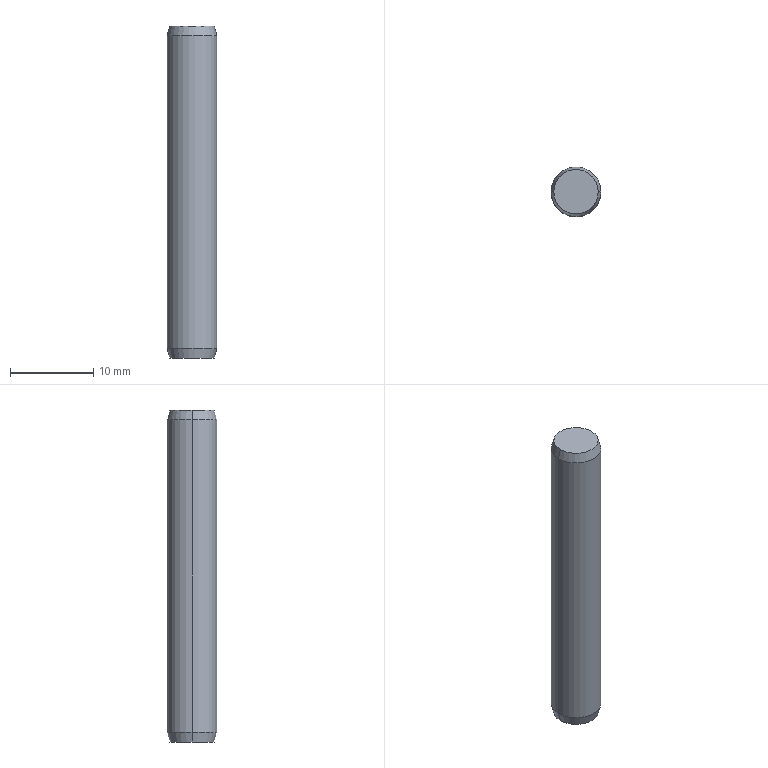Component | NX | GB_T_119_1_2000_CYLINDRICALPIN_6X40 | 1 solid | 8 faces | box 6 x 6 x 40 mm | volume 1124 mm3 | cone 4 | cylinder 2 | plane 2 | commonest cylinder face diameters 6 x2
STEP:
#1=CARTESIAN_POINT('',(0.,0.,0.));
#2=DIRECTION('',(0.,0.,1.));
#3=DIRECTION('',(1.,0.,0.));
#4=AXIS2_PLACEMENT_3D('',#1,#2,#3);
#5=CARTESIAN_POINT('',(7.514,-108.,34.));
#6=VERTEX_POINT('',#5);
#7=CARTESIAN_POINT('',(2.157,-108.,34.));
#8=VERTEX_POINT('',#7);
#9=CARTESIAN_POINT('',(4.835,-108.,34.));
#10=DIRECTION('',(0.,0.,1.));
#11=DIRECTION('',(1.,0.,0.));
#12=AXIS2_PLACEMENT_3D('',#9,#10,#11);
#13=CIRCLE('',#12,2.678);
#14=CARTESIAN_POINT('',(4.835,-108.,35.2));
#15=DIRECTION('',(0.,0.,1.));
#16=DIRECTION('',(-1.,0.,0.));
#17=AXIS2_PLACEMENT_3D('',#14,#15,#16);
#18=CONICAL_SURFACE('',#17,3.,0.2618);
#19=CARTESIAN_POINT('',(3.142,-1.2));
#20=DIRECTION('',(1.,0.));
#21=VECTOR('',#20,1.);
#22=LINE('',#19,#21);
#23=(GEOMETRIC_REPRESENTATION_CONTEXT(2)PARAMETRIC_REPRESENTATION_CONTEXT()REPRESENTATION_CONTEXT('',''));
#24=DEFINITIONAL_REPRESENTATION('',(#22),#23);
#25=PCURVE('',#18,#24);
#26=CARTESIAN_POINT('',(4.835,-105.322,34.));
#27=DIRECTION('',(0.,0.,-1.));
#28=DIRECTION('',(1.,0.,0.));
#29=AXIS2_PLACEMENT_3D('',#26,#27,#28);
#30=PLANE('',#29);
#31=CARTESIAN_POINT('',(2.678,2.678));
#32=CARTESIAN_POINT('',(2.678,-1.961));
#33=CARTESIAN_POINT('',(-1.339,0.3588));
#34=CARTESIAN_POINT('',(-5.357,2.678));
#35=CARTESIAN_POINT('',(-1.339,4.998));
#36=CARTESIAN_POINT('',(2.678,7.318));
#37=CARTESIAN_POINT('',(2.678,2.678));
#38=(BOUNDED_CURVE()B_SPLINE_CURVE(2,(#31,#32,#33,#34,#35,#36,#37),.UNSPECIFIED.,.T.,.F.)B_SPLINE_CURVE_WITH_KNOTS((1,2,2,2,2,1),(-2.094,0.,2.094,4.189,6.283,8.378),.UNSPECIFIED.)CURVE()GEOMETRIC_REPRESENTATION_ITEM()RATIONAL_B_SPLINE_CURVE((1.,0.5,1.,0.5,1.,0.5,1.))REPRESENTATION_ITEM(''));
#39=(GEOMETRIC_REPRESENTATION_CONTEXT(2)PARAMETRIC_REPRESENTATION_CONTEXT()REPRESENTATION_CONTEXT('',''));
#40=DEFINITIONAL_REPRESENTATION('',(#38),#39);
#41=PCURVE('',#30,#40);
#42=SURFACE_CURVE('',#13,(#25,#41),.PCURVE_S1.);
#43=EDGE_CURVE('',#6,#8,#42,.T.);
#44=ORIENTED_EDGE('',*,*,#43,.T.);
#45=CARTESIAN_POINT('',(1.835,-108.,35.2));
#46=VERTEX_POINT('',#45);
#47=CARTESIAN_POINT('',(1.835,-108.,35.2));
#48=DIRECTION('',(-0.2588,0.,0.9659));
#49=VECTOR('',#48,1.);
#50=LINE('',#47,#49);
#51=CARTESIAN_POINT('',(6.283,-0.));
#52=DIRECTION('',(0.,1.));
#53=VECTOR('',#52,1.);
#54=LINE('',#51,#53);
#55=(GEOMETRIC_REPRESENTATION_CONTEXT(2)PARAMETRIC_REPRESENTATION_CONTEXT()REPRESENTATION_CONTEXT('',''));
#56=DEFINITIONAL_REPRESENTATION('',(#54),#55);
#57=PCURVE('',#18,#56);
#58=CARTESIAN_POINT('',(4.835,-108.,35.2));
#59=DIRECTION('',(0.,0.,1.));
#60=DIRECTION('',(-1.,0.,0.));
#61=AXIS2_PLACEMENT_3D('',#58,#59,#60);
#62=CONICAL_SURFACE('',#61,3.,0.2618);
#63=CARTESIAN_POINT('',(0.,-0.));
#64=DIRECTION('',(0.,1.));
#65=VECTOR('',#64,1.);
#66=LINE('',#63,#65);
#67=(GEOMETRIC_REPRESENTATION_CONTEXT(2)PARAMETRIC_REPRESENTATION_CONTEXT()REPRESENTATION_CONTEXT('',''));
#68=DEFINITIONAL_REPRESENTATION('',(#66),#67);
#69=PCURVE('',#62,#68);
#70=SURFACE_CURVE('',#50,(#57,#69),.PCURVE_S1.);
#71=EDGE_CURVE('',#8,#46,#70,.T.);
#72=ORIENTED_EDGE('',*,*,#71,.T.);
#73=CARTESIAN_POINT('',(7.835,-108.,35.2));
#74=VERTEX_POINT('',#73);
#75=CARTESIAN_POINT('',(4.835,-108.,35.2));
#76=DIRECTION('',(0.,0.,1.));
#77=DIRECTION('',(1.,0.,0.));
#78=AXIS2_PLACEMENT_3D('',#75,#76,#77);
#79=CIRCLE('',#78,3.);
#80=CARTESIAN_POINT('',(3.142,0.));
#81=DIRECTION('',(1.,0.));
#82=VECTOR('',#81,1.);
#83=LINE('',#80,#82);
#84=(GEOMETRIC_REPRESENTATION_CONTEXT(2)PARAMETRIC_REPRESENTATION_CONTEXT()REPRESENTATION_CONTEXT('',''));
#85=DEFINITIONAL_REPRESENTATION('',(#83),#84);
#86=PCURVE('',#18,#85);
#87=CARTESIAN_POINT('',(4.835,-108.,34.));
#88=DIRECTION('',(0.,0.,1.));
#89=DIRECTION('',(-1.,0.,0.));
#90=AXIS2_PLACEMENT_3D('',#87,#88,#89);
#91=CYLINDRICAL_SURFACE('',#90,3.);
#92=CARTESIAN_POINT('',(3.142,1.2));
#93=DIRECTION('',(1.,0.));
#94=VECTOR('',#93,1.);
#95=LINE('',#92,#94);
#96=(GEOMETRIC_REPRESENTATION_CONTEXT(2)PARAMETRIC_REPRESENTATION_CONTEXT()REPRESENTATION_CONTEXT('',''));
#97=DEFINITIONAL_REPRESENTATION('',(#95),#96);
#98=PCURVE('',#91,#97);
#99=SURFACE_CURVE('',#79,(#86,#98),.PCURVE_S1.);
#100=EDGE_CURVE('',#74,#46,#99,.T.);
#101=ORIENTED_EDGE('',*,*,#100,.F.);
#102=CARTESIAN_POINT('',(7.835,-108.,35.2));
#103=DIRECTION('',(0.2588,0.,0.9659));
#104=VECTOR('',#103,1.);
#105=LINE('',#102,#104);
#106=CARTESIAN_POINT('',(3.142,-0.));
#107=DIRECTION('',(0.,1.));
#108=VECTOR('',#107,1.);
#109=LINE('',#106,#108);
#110=(GEOMETRIC_REPRESENTATION_CONTEXT(2)PARAMETRIC_REPRESENTATION_CONTEXT()REPRESENTATION_CONTEXT('',''));
#111=DEFINITIONAL_REPRESENTATION('',(#109),#110);
#112=PCURVE('',#18,#111);
#113=CARTESIAN_POINT('',(3.142,-0.));
#114=DIRECTION('',(0.,1.));
#115=VECTOR('',#114,1.);
#116=LINE('',#113,#115);
#117=(GEOMETRIC_REPRESENTATION_CONTEXT(2)PARAMETRIC_REPRESENTATION_CONTEXT()REPRESENTATION_CONTEXT('',''));
#118=DEFINITIONAL_REPRESENTATION('',(#116),#117);
#119=PCURVE('',#62,#118);
#120=SURFACE_CURVE('',#105,(#112,#119),.PCURVE_S1.);
#121=EDGE_CURVE('',#6,#74,#120,.T.);
#122=ORIENTED_EDGE('',*,*,#121,.F.);
#123=EDGE_LOOP('',(#44,#72,#101,#122));
#124=FACE_BOUND('',#123,.T.);
#125=ADVANCED_FACE('',(#124),#18,.T.);
#126=ORIENTED_EDGE('',*,*,#100,.T.);
#127=CARTESIAN_POINT('',(1.835,-108.,72.8));
#128=VERTEX_POINT('',#127);
#129=CARTESIAN_POINT('',(1.835,-108.,34.));
#130=DIRECTION('',(0.,0.,1.));
#131=VECTOR('',#130,1.);
#132=LINE('',#129,#131);
#133=CARTESIAN_POINT('',(6.283,0.));
#134=DIRECTION('',(0.,1.));
#135=VECTOR('',#134,1.);
#136=LINE('',#133,#135);
#137=(GEOMETRIC_REPRESENTATION_CONTEXT(2)PARAMETRIC_REPRESENTATION_CONTEXT()REPRESENTATION_CONTEXT('',''));
#138=DEFINITIONAL_REPRESENTATION('',(#136),#137);
#139=PCURVE('',#91,#138);
#140=CARTESIAN_POINT('',(4.835,-108.,34.));
#141=DIRECTION('',(0.,0.,1.));
#142=DIRECTION('',(-1.,0.,0.));
#143=AXIS2_PLACEMENT_3D('',#140,#141,#142);
#144=CYLINDRICAL_SURFACE('',#143,3.);
#145=CARTESIAN_POINT('',(0.,0.));
#146=DIRECTION('',(0.,1.));
#147=VECTOR('',#146,1.);
#148=LINE('',#145,#147);
#149=(GEOMETRIC_REPRESENTATION_CONTEXT(2)PARAMETRIC_REPRESENTATION_CONTEXT()REPRESENTATION_CONTEXT('',''));
#150=DEFINITIONAL_REPRESENTATION('',(#148),#149);
#151=PCURVE('',#144,#150);
#152=SURFACE_CURVE('',#132,(#139,#151),.PCURVE_S1.);
#153=EDGE_CURVE('',#46,#128,#152,.T.);
#154=ORIENTED_EDGE('',*,*,#153,.T.);
#155=CARTESIAN_POINT('',(7.835,-108.,72.8));
#156=VERTEX_POINT('',#155);
#157=CARTESIAN_POINT('',(4.835,-108.,72.8));
#158=DIRECTION('',(0.,0.,1.));
#159=DIRECTION('',(1.,0.,0.));
#160=AXIS2_PLACEMENT_3D('',#157,#158,#159);
#161=CIRCLE('',#160,3.);
#162=CARTESIAN_POINT('',(3.142,38.8));
#163=DIRECTION('',(1.,0.));
#164=VECTOR('',#163,1.);
#165=LINE('',#162,#164);
#166=(GEOMETRIC_REPRESENTATION_CONTEXT(2)PARAMETRIC_REPRESENTATION_CONTEXT()REPRESENTATION_CONTEXT('',''));
#167=DEFINITIONAL_REPRESENTATION('',(#165),#166);
#168=PCURVE('',#91,#167);
#169=CARTESIAN_POINT('',(4.835,-108.,74.));
#170=DIRECTION('',(0.,0.,-1.));
#171=DIRECTION('',(1.,0.,0.));
#172=AXIS2_PLACEMENT_3D('',#169,#170,#171);
#173=CONICAL_SURFACE('',#172,2.678,0.2618);
#174=CARTESIAN_POINT('',(6.283,1.2));
#175=DIRECTION('',(-1.,0.));
#176=VECTOR('',#175,1.);
#177=LINE('',#174,#176);
#178=(GEOMETRIC_REPRESENTATION_CONTEXT(2)PARAMETRIC_REPRESENTATION_CONTEXT()REPRESENTATION_CONTEXT('',''));
#179=DEFINITIONAL_REPRESENTATION('',(#177),#178);
#180=PCURVE('',#173,#179);
#181=SURFACE_CURVE('',#161,(#168,#180),.PCURVE_S1.);
#182=EDGE_CURVE('',#156,#128,#181,.T.);
#183=ORIENTED_EDGE('',*,*,#182,.F.);
#184=CARTESIAN_POINT('',(7.835,-108.,34.));
#185=DIRECTION('',(0.,0.,1.));
#186=VECTOR('',#185,1.);
#187=LINE('',#184,#186);
#188=CARTESIAN_POINT('',(3.142,0.));
#189=DIRECTION('',(0.,1.));
#190=VECTOR('',#189,1.);
#191=LINE('',#188,#190);
#192=(GEOMETRIC_REPRESENTATION_CONTEXT(2)PARAMETRIC_REPRESENTATION_CONTEXT()REPRESENTATION_CONTEXT('',''));
#193=DEFINITIONAL_REPRESENTATION('',(#191),#192);
#194=PCURVE('',#91,#193);
#195=CARTESIAN_POINT('',(3.142,0.));
#196=DIRECTION('',(0.,1.));
#197=VECTOR('',#196,1.);
#198=LINE('',#195,#197);
#199=(GEOMETRIC_REPRESENTATION_CONTEXT(2)PARAMETRIC_REPRESENTATION_CONTEXT()REPRESENTATION_CONTEXT('',''));
#200=DEFINITIONAL_REPRESENTATION('',(#198),#199);
#201=PCURVE('',#144,#200);
#202=SURFACE_CURVE('',#187,(#194,#201),.PCURVE_S1.);
#203=EDGE_CURVE('',#74,#156,#202,.T.);
#204=ORIENTED_EDGE('',*,*,#203,.F.);
#205=EDGE_LOOP('',(#126,#154,#183,#204));
#206=FACE_BOUND('',#205,.T.);
#207=ADVANCED_FACE('',(#206),#91,.T.);
#208=CARTESIAN_POINT('',(7.514,-108.,74.));
#209=VERTEX_POINT('',#208);
#210=CARTESIAN_POINT('',(2.157,-108.,74.));
#211=VERTEX_POINT('',#210);
#212=CARTESIAN_POINT('',(4.835,-108.,74.));
#213=DIRECTION('',(0.,0.,1.));
#214=DIRECTION('',(1.,0.,0.));
#215=AXIS2_PLACEMENT_3D('',#212,#213,#214);
#216=CIRCLE('',#215,2.678);
#217=CARTESIAN_POINT('',(6.283,0.));
#218=DIRECTION('',(-1.,0.));
#219=VECTOR('',#218,1.);
#220=LINE('',#217,#219);
#221=(GEOMETRIC_REPRESENTATION_CONTEXT(2)PARAMETRIC_REPRESENTATION_CONTEXT()REPRESENTATION_CONTEXT('',''));
#222=DEFINITIONAL_REPRESENTATION('',(#220),#221);
#223=PCURVE('',#173,#222);
#224=CARTESIAN_POINT('',(4.835,-105.322,74.));
#225=DIRECTION('',(0.,0.,1.));
#226=DIRECTION('',(-1.,0.,0.));
#227=AXIS2_PLACEMENT_3D('',#224,#225,#226);
#228=PLANE('',#227);
#229=CARTESIAN_POINT('',(0.,2.678));
#230=DIRECTION('',(-1.,0.));
#231=AXIS2_PLACEMENT_2D('',#229,#230);
#232=CIRCLE('',#231,2.678);
#233=(GEOMETRIC_REPRESENTATION_CONTEXT(2)PARAMETRIC_REPRESENTATION_CONTEXT()REPRESENTATION_CONTEXT('',''));
#234=DEFINITIONAL_REPRESENTATION('',(#232),#233);
#235=PCURVE('',#228,#234);
#236=SURFACE_CURVE('',#216,(#223,#235),.PCURVE_S1.);
#237=EDGE_CURVE('',#209,#211,#236,.T.);
#238=ORIENTED_EDGE('',*,*,#237,.F.);
#239=CARTESIAN_POINT('',(7.514,-108.,74.));
#240=DIRECTION('',(0.2588,0.,-0.9659));
#241=VECTOR('',#240,1.);
#242=LINE('',#239,#241);
#243=CARTESIAN_POINT('',(6.283,-0.));
#244=DIRECTION('',(0.,1.));
#245=VECTOR('',#244,1.);
#246=LINE('',#243,#245);
#247=(GEOMETRIC_REPRESENTATION_CONTEXT(2)PARAMETRIC_REPRESENTATION_CONTEXT()REPRESENTATION_CONTEXT('',''));
#248=DEFINITIONAL_REPRESENTATION('',(#246),#247);
#249=PCURVE('',#173,#248);
#250=CARTESIAN_POINT('',(4.835,-108.,74.));
#251=DIRECTION('',(0.,0.,-1.));
#252=DIRECTION('',(1.,0.,0.));
#253=AXIS2_PLACEMENT_3D('',#250,#251,#252);
#254=CONICAL_SURFACE('',#253,2.678,0.2618);
#255=CARTESIAN_POINT('',(0.,-0.));
#256=DIRECTION('',(0.,1.));
#257=VECTOR('',#256,1.);
#258=LINE('',#255,#257);
#259=(GEOMETRIC_REPRESENTATION_CONTEXT(2)PARAMETRIC_REPRESENTATION_CONTEXT()REPRESENTATION_CONTEXT('',''));
#260=DEFINITIONAL_REPRESENTATION('',(#258),#259);
#261=PCURVE('',#254,#260);
#262=SURFACE_CURVE('',#242,(#249,#261),.PCURVE_S1.);
#263=EDGE_CURVE('',#209,#156,#262,.T.);
#264=ORIENTED_EDGE('',*,*,#263,.T.);
#265=ORIENTED_EDGE('',*,*,#182,.T.);
#266=CARTESIAN_POINT('',(2.157,-108.,74.));
#267=DIRECTION('',(-0.2588,0.,-0.9659));
#268=VECTOR('',#267,1.);
#269=LINE('',#266,#268);
#270=CARTESIAN_POINT('',(3.142,0.));
#271=DIRECTION('',(0.,1.));
#272=VECTOR('',#271,1.);
#273=LINE('',#270,#272);
#274=(GEOMETRIC_REPRESENTATION_CONTEXT(2)PARAMETRIC_REPRESENTATION_CONTEXT()REPRESENTATION_CONTEXT('',''));
#275=DEFINITIONAL_REPRESENTATION('',(#273),#274);
#276=PCURVE('',#173,#275);
#277=CARTESIAN_POINT('',(3.142,0.));
#278=DIRECTION('',(0.,1.));
#279=VECTOR('',#278,1.);
#280=LINE('',#277,#279);
#281=(GEOMETRIC_REPRESENTATION_CONTEXT(2)PARAMETRIC_REPRESENTATION_CONTEXT()REPRESENTATION_CONTEXT('',''));
#282=DEFINITIONAL_REPRESENTATION('',(#280),#281);
#283=PCURVE('',#254,#282);
#284=SURFACE_CURVE('',#269,(#276,#283),.PCURVE_S1.);
#285=EDGE_CURVE('',#211,#128,#284,.T.);
#286=ORIENTED_EDGE('',*,*,#285,.F.);
#287=EDGE_LOOP('',(#238,#264,#265,#286));
#288=FACE_BOUND('',#287,.T.);
#289=ADVANCED_FACE('',(#288),#173,.T.);
#290=ORIENTED_EDGE('',*,*,#43,.F.);
#291=CARTESIAN_POINT('',(4.835,-108.,34.));
#292=DIRECTION('',(0.,0.,1.));
#293=DIRECTION('',(1.,0.,0.));
#294=AXIS2_PLACEMENT_3D('',#291,#292,#293);
#295=CIRCLE('',#294,2.678);
#296=CARTESIAN_POINT('',(2.678,2.678));
#297=CARTESIAN_POINT('',(2.678,-1.961));
#298=CARTESIAN_POINT('',(-1.339,0.3588));
#299=CARTESIAN_POINT('',(-5.357,2.678));
#300=CARTESIAN_POINT('',(-1.339,4.998));
#301=CARTESIAN_POINT('',(2.678,7.318));
#302=CARTESIAN_POINT('',(2.678,2.678));
#303=(BOUNDED_CURVE()B_SPLINE_CURVE(2,(#296,#297,#298,#299,#300,#301,#302),.UNSPECIFIED.,.T.,.F.)B_SPLINE_CURVE_WITH_KNOTS((1,2,2,2,2,1),(-2.094,0.,2.094,4.189,6.283,8.378),.UNSPECIFIED.)CURVE()GEOMETRIC_REPRESENTATION_ITEM()RATIONAL_B_SPLINE_CURVE((1.,0.5,1.,0.5,1.,0.5,1.))REPRESENTATION_ITEM(''));
#304=(GEOMETRIC_REPRESENTATION_CONTEXT(2)PARAMETRIC_REPRESENTATION_CONTEXT()REPRESENTATION_CONTEXT('',''));
#305=DEFINITIONAL_REPRESENTATION('',(#303),#304);
#306=PCURVE('',#30,#305);
#307=CARTESIAN_POINT('',(-3.142,-1.2));
#308=DIRECTION('',(1.,0.));
#309=VECTOR('',#308,1.);
#310=LINE('',#307,#309);
#311=(GEOMETRIC_REPRESENTATION_CONTEXT(2)PARAMETRIC_REPRESENTATION_CONTEXT()REPRESENTATION_CONTEXT('',''));
#312=DEFINITIONAL_REPRESENTATION('',(#310),#311);
#313=PCURVE('',#62,#312);
#314=SURFACE_CURVE('',#295,(#306,#313),.PCURVE_S1.);
#315=EDGE_CURVE('',#8,#6,#314,.T.);
#316=ORIENTED_EDGE('',*,*,#315,.F.);
#317=EDGE_LOOP('',(#290,#316));
#318=FACE_BOUND('',#317,.T.);
#319=ADVANCED_FACE('',(#318),#30,.T.);
#320=CARTESIAN_POINT('',(4.835,-108.,74.));
#321=DIRECTION('',(0.,0.,1.));
#322=DIRECTION('',(1.,0.,0.));
#323=AXIS2_PLACEMENT_3D('',#320,#321,#322);
#324=CIRCLE('',#323,2.678);
#325=CARTESIAN_POINT('',(0.,2.678));
#326=DIRECTION('',(-1.,0.));
#327=AXIS2_PLACEMENT_2D('',#325,#326);
#328=CIRCLE('',#327,2.678);
#329=(GEOMETRIC_REPRESENTATION_CONTEXT(2)PARAMETRIC_REPRESENTATION_CONTEXT()REPRESENTATION_CONTEXT('',''));
#330=DEFINITIONAL_REPRESENTATION('',(#328),#329);
#331=PCURVE('',#228,#330);
#332=CARTESIAN_POINT('',(6.283,0.));
#333=DIRECTION('',(-1.,0.));
#334=VECTOR('',#333,1.);
#335=LINE('',#332,#334);
#336=(GEOMETRIC_REPRESENTATION_CONTEXT(2)PARAMETRIC_REPRESENTATION_CONTEXT()REPRESENTATION_CONTEXT('',''));
#337=DEFINITIONAL_REPRESENTATION('',(#335),#336);
#338=PCURVE('',#254,#337);
#339=SURFACE_CURVE('',#324,(#331,#338),.PCURVE_S1.);
#340=EDGE_CURVE('',#211,#209,#339,.T.);
#341=ORIENTED_EDGE('',*,*,#340,.T.);
#342=ORIENTED_EDGE('',*,*,#237,.T.);
#343=EDGE_LOOP('',(#341,#342));
#344=FACE_BOUND('',#343,.T.);
#345=ADVANCED_FACE('',(#344),#228,.T.);
#346=ORIENTED_EDGE('',*,*,#263,.F.);
#347=ORIENTED_EDGE('',*,*,#340,.F.);
#348=ORIENTED_EDGE('',*,*,#285,.T.);
#349=CARTESIAN_POINT('',(4.835,-108.,72.8));
#350=DIRECTION('',(0.,0.,1.));
#351=DIRECTION('',(1.,0.,0.));
#352=AXIS2_PLACEMENT_3D('',#349,#350,#351);
#353=CIRCLE('',#352,3.);
#354=CARTESIAN_POINT('',(6.283,1.2));
#355=DIRECTION('',(-1.,0.));
#356=VECTOR('',#355,1.);
#357=LINE('',#354,#356);
#358=(GEOMETRIC_REPRESENTATION_CONTEXT(2)PARAMETRIC_REPRESENTATION_CONTEXT()REPRESENTATION_CONTEXT('',''));
#359=DEFINITIONAL_REPRESENTATION('',(#357),#358);
#360=PCURVE('',#254,#359);
#361=CARTESIAN_POINT('',(-3.142,38.8));
#362=DIRECTION('',(1.,0.));
#363=VECTOR('',#362,1.);
#364=LINE('',#361,#363);
#365=(GEOMETRIC_REPRESENTATION_CONTEXT(2)PARAMETRIC_REPRESENTATION_CONTEXT()REPRESENTATION_CONTEXT('',''));
#366=DEFINITIONAL_REPRESENTATION('',(#364),#365);
#367=PCURVE('',#144,#366);
#368=SURFACE_CURVE('',#353,(#360,#367),.PCURVE_S1.);
#369=EDGE_CURVE('',#128,#156,#368,.T.);
#370=ORIENTED_EDGE('',*,*,#369,.T.);
#371=EDGE_LOOP('',(#346,#347,#348,#370));
#372=FACE_BOUND('',#371,.T.);
#373=ADVANCED_FACE('',(#372),#254,.T.);
#374=ORIENTED_EDGE('',*,*,#153,.F.);
#375=CARTESIAN_POINT('',(4.835,-108.,35.2));
#376=DIRECTION('',(0.,0.,1.));
#377=DIRECTION('',(1.,0.,0.));
#378=AXIS2_PLACEMENT_3D('',#375,#376,#377);
#379=CIRCLE('',#378,3.);
#380=CARTESIAN_POINT('',(-3.142,1.2));
#381=DIRECTION('',(1.,0.));
#382=VECTOR('',#381,1.);
#383=LINE('',#380,#382);
#384=(GEOMETRIC_REPRESENTATION_CONTEXT(2)PARAMETRIC_REPRESENTATION_CONTEXT()REPRESENTATION_CONTEXT('',''));
#385=DEFINITIONAL_REPRESENTATION('',(#383),#384);
#386=PCURVE('',#144,#385);
#387=CARTESIAN_POINT('',(-3.142,0.));
#388=DIRECTION('',(1.,0.));
#389=VECTOR('',#388,1.);
#390=LINE('',#387,#389);
#391=(GEOMETRIC_REPRESENTATION_CONTEXT(2)PARAMETRIC_REPRESENTATION_CONTEXT()REPRESENTATION_CONTEXT('',''));
#392=DEFINITIONAL_REPRESENTATION('',(#390),#391);
#393=PCURVE('',#62,#392);
#394=SURFACE_CURVE('',#379,(#386,#393),.PCURVE_S1.);
#395=EDGE_CURVE('',#46,#74,#394,.T.);
#396=ORIENTED_EDGE('',*,*,#395,.T.);
#397=ORIENTED_EDGE('',*,*,#203,.T.);
#398=ORIENTED_EDGE('',*,*,#369,.F.);
#399=EDGE_LOOP('',(#374,#396,#397,#398));
#400=FACE_BOUND('',#399,.T.);
#401=ADVANCED_FACE('',(#400),#144,.T.);
#402=ORIENTED_EDGE('',*,*,#71,.F.);
#403=ORIENTED_EDGE('',*,*,#315,.T.);
#404=ORIENTED_EDGE('',*,*,#121,.T.);
#405=ORIENTED_EDGE('',*,*,#395,.F.);
#406=EDGE_LOOP('',(#402,#403,#404,#405));
#407=FACE_BOUND('',#406,.T.);
#408=ADVANCED_FACE('',(#407),#62,.T.);
#409=CLOSED_SHELL('',(#125,#207,#289,#319,#345,#373,#401,#408));
#410=MANIFOLD_SOLID_BREP('',#409);
#411=(LENGTH_UNIT()NAMED_UNIT(*)SI_UNIT(.MILLI.,.METRE.));
#412=UNCERTAINTY_MEASURE_WITH_UNIT(LENGTH_MEASURE(0.0000001),#411,'','');
#413=(NAMED_UNIT(*)PLANE_ANGLE_UNIT()SI_UNIT($,.RADIAN.));
#414=(NAMED_UNIT(*)SI_UNIT($,.STERADIAN.)SOLID_ANGLE_UNIT());
#415=(GEOMETRIC_REPRESENTATION_CONTEXT(3)GLOBAL_UNCERTAINTY_ASSIGNED_CONTEXT((#412))GLOBAL_UNIT_ASSIGNED_CONTEXT((#411,#413,#414))REPRESENTATION_CONTEXT('',''));
#416=ADVANCED_BREP_SHAPE_REPRESENTATION('',(#4,#410),#415);